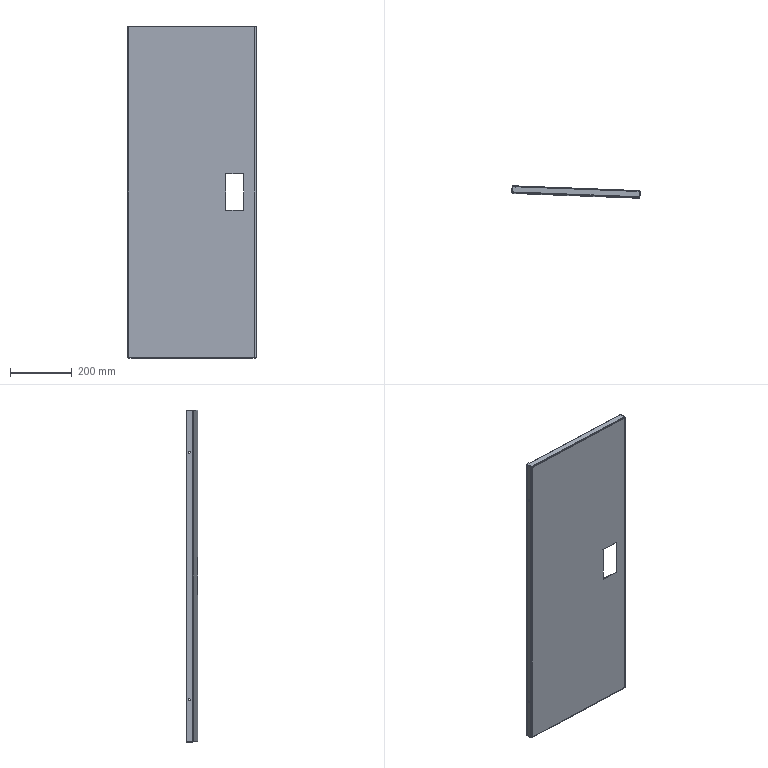Component | SolidWorks | DoorPanel415-1 | 1 solid | 94 faces | volume 783364 mm3 | plane 66 | cylinder 20 | spline 8 | commonest cylinder face diameters 6 x8 3 x8 7 x4